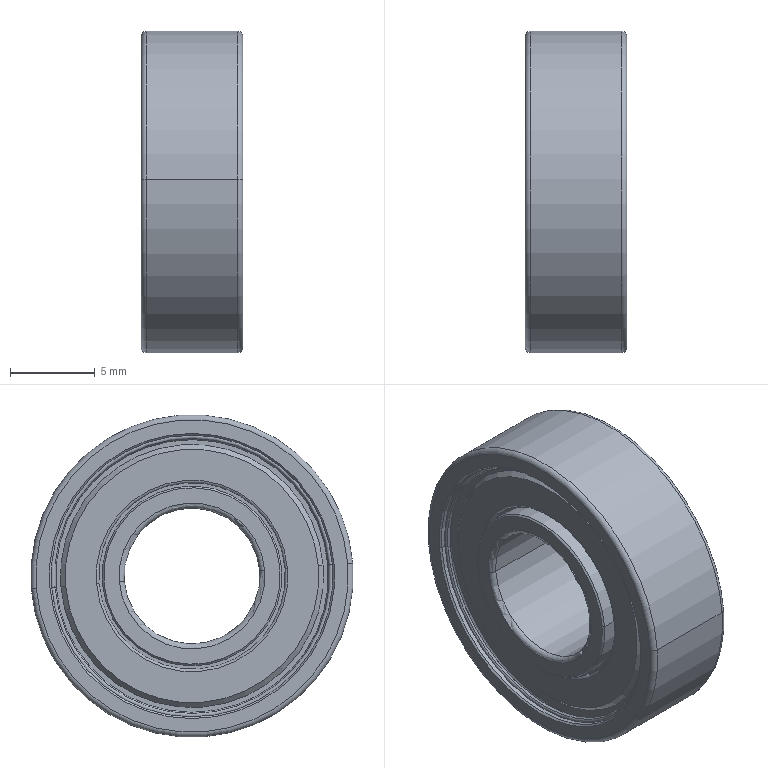Component | SolidWorks | BAF698ZZ-SUS.stp-13 | 1 solid | 108 faces | volume 1044 mm3 | cone 40 | cylinder 28 | torus 24 | plane 16 | commonest cylinder face diameters 11.5 x4 15.5 x4 11.284 x4 11 x4 16.6 x4 10.6 x4 19 x2 8 x2 | material AISI 304